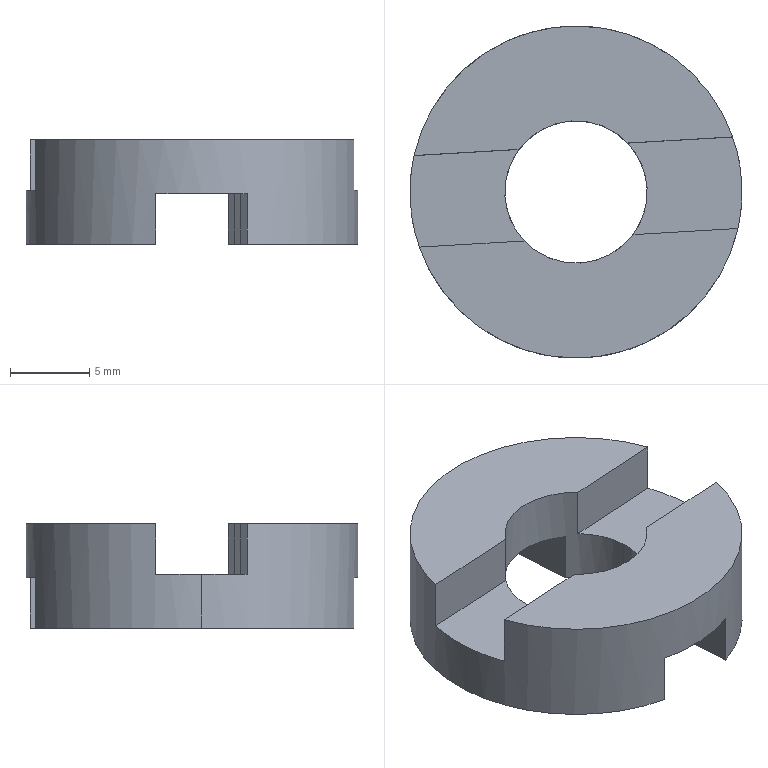Component | SolidWorks | MotorAssemblyWhen2-1_MCOCG20-8-10-1_MCOCG_spacer22-1 | 1 solid | 20 faces | box 21 x 21 x 6.6 mm | volume 1406 mm3 | plane 16 | cylinder 4 | commonest cylinder face diameters 21 x2 9 x2
STEP:
#1=COLOUR_RGB('',0.7922,0.8196,0.9333);
#2=FILL_AREA_STYLE_COLOUR('',#1);
#3=FILL_AREA_STYLE('',(#2));
#4=SURFACE_STYLE_FILL_AREA(#3);
#5=SURFACE_SIDE_STYLE('',(#4));
#6=SURFACE_STYLE_USAGE(.BOTH.,#5);
#7=PRESENTATION_STYLE_ASSIGNMENT((#6));
#8=CARTESIAN_POINT('',(-1.831,4.945,-4.699));
#9=VERTEX_POINT('',#8);
#10=CARTESIAN_POINT('',(-1.556,5.359,-4.699));
#11=VERTEX_POINT('',#10);
#12=CARTESIAN_POINT('',(-1.969,5.335,-4.699));
#13=DIRECTION('',(0.,-0.,1.));
#14=DIRECTION('',(-0.9983,-0.05821,0.));
#15=AXIS2_PLACEMENT_3D('',#12,#13,#14);
#16=CIRCLE('',#15,0.4134);
#17=EDGE_CURVE('',#9,#11,#16,.T.);
#18=ORIENTED_EDGE('',*,*,#17,.T.);
#19=CARTESIAN_POINT('',(-1.556,5.359,-4.565));
#20=VERTEX_POINT('',#19);
#21=CARTESIAN_POINT('',(-1.556,5.359,-4.699));
#22=DIRECTION('',(0.,-0.,1.));
#23=VECTOR('',#22,39.37);
#24=LINE('',#21,#23);
#25=EDGE_CURVE('',#11,#20,#24,.T.);
#26=ORIENTED_EDGE('',*,*,#25,.T.);
#27=CARTESIAN_POINT('',(-1.565,5.244,-4.565));
#28=VERTEX_POINT('',#27);
#29=CARTESIAN_POINT('',(-1.969,5.335,-4.565));
#30=DIRECTION('',(-0.,0.,-1.));
#31=DIRECTION('',(-0.9983,-0.05821,0.));
#32=AXIS2_PLACEMENT_3D('',#29,#30,#31);
#33=CIRCLE('',#32,0.4134);
#34=EDGE_CURVE('',#20,#28,#33,.T.);
#35=ORIENTED_EDGE('',*,*,#34,.T.);
#36=CARTESIAN_POINT('',(-1.565,5.244,-4.439));
#37=VERTEX_POINT('',#36);
#38=CARTESIAN_POINT('',(-1.565,5.244,-4.699));
#39=DIRECTION('',(0.,-0.,1.));
#40=VECTOR('',#39,39.37);
#41=LINE('',#38,#40);
#42=EDGE_CURVE('',#28,#37,#41,.T.);
#43=ORIENTED_EDGE('',*,*,#42,.T.);
#44=CARTESIAN_POINT('',(-2.358,5.198,-4.439));
#45=VERTEX_POINT('',#44);
#46=CARTESIAN_POINT('',(-1.969,5.335,-4.439));
#47=DIRECTION('',(-0.,0.,-1.));
#48=DIRECTION('',(-0.9983,-0.05821,0.));
#49=AXIS2_PLACEMENT_3D('',#46,#47,#48);
#50=CIRCLE('',#49,0.4134);
#51=EDGE_CURVE('',#37,#45,#50,.T.);
#52=ORIENTED_EDGE('',*,*,#51,.T.);
#53=CARTESIAN_POINT('',(-2.358,5.198,-4.565));
#54=VERTEX_POINT('',#53);
#55=CARTESIAN_POINT('',(-2.358,5.198,-4.699));
#56=DIRECTION('',(-0.,0.,-1.));
#57=VECTOR('',#56,39.37);
#58=LINE('',#55,#57);
#59=EDGE_CURVE('',#45,#54,#58,.T.);
#60=ORIENTED_EDGE('',*,*,#59,.T.);
#61=CARTESIAN_POINT('',(-2.381,5.311,-4.565));
#62=VERTEX_POINT('',#61);
#63=CARTESIAN_POINT('',(-1.969,5.335,-4.565));
#64=DIRECTION('',(-0.,0.,-1.));
#65=DIRECTION('',(-0.9983,-0.05821,0.));
#66=AXIS2_PLACEMENT_3D('',#63,#64,#65);
#67=CIRCLE('',#66,0.4134);
#68=EDGE_CURVE('',#54,#62,#67,.T.);
#69=ORIENTED_EDGE('',*,*,#68,.T.);
#70=CARTESIAN_POINT('',(-2.381,5.311,-4.699));
#71=VERTEX_POINT('',#70);
#72=CARTESIAN_POINT('',(-2.381,5.311,-4.699));
#73=DIRECTION('',(0.,-0.,1.));
#74=VECTOR('',#73,39.37);
#75=LINE('',#72,#74);
#76=EDGE_CURVE('',#71,#62,#75,.T.);
#77=ORIENTED_EDGE('',*,*,#76,.F.);
#78=CARTESIAN_POINT('',(-2.059,4.931,-4.699));
#79=VERTEX_POINT('',#78);
#80=CARTESIAN_POINT('',(-1.969,5.335,-4.699));
#81=DIRECTION('',(0.,-0.,1.));
#82=DIRECTION('',(-0.9983,-0.05821,0.));
#83=AXIS2_PLACEMENT_3D('',#80,#81,#82);
#84=CIRCLE('',#83,0.4134);
#85=EDGE_CURVE('',#71,#79,#84,.T.);
#86=ORIENTED_EDGE('',*,*,#85,.T.);
#87=CARTESIAN_POINT('',(-2.059,4.931,-4.573));
#88=VERTEX_POINT('',#87);
#89=CARTESIAN_POINT('',(-2.059,4.931,-4.699));
#90=DIRECTION('',(0.,-0.,1.));
#91=VECTOR('',#90,39.37);
#92=LINE('',#89,#91);
#93=EDGE_CURVE('',#79,#88,#92,.T.);
#94=ORIENTED_EDGE('',*,*,#93,.T.);
#95=CARTESIAN_POINT('',(-1.831,4.945,-4.573));
#96=VERTEX_POINT('',#95);
#97=CARTESIAN_POINT('',(-1.969,5.335,-4.573));
#98=DIRECTION('',(0.,-0.,1.));
#99=DIRECTION('',(-0.9983,-0.05821,0.));
#100=AXIS2_PLACEMENT_3D('',#97,#98,#99);
#101=CIRCLE('',#100,0.4134);
#102=EDGE_CURVE('',#88,#96,#101,.T.);
#103=ORIENTED_EDGE('',*,*,#102,.T.);
#104=CARTESIAN_POINT('',(-1.831,4.945,-4.699));
#105=DIRECTION('',(-0.,0.,-1.));
#106=VECTOR('',#105,39.37);
#107=LINE('',#104,#106);
#108=EDGE_CURVE('',#96,#9,#107,.T.);
#109=ORIENTED_EDGE('',*,*,#108,.T.);
#110=EDGE_LOOP('',(#18,#26,#35,#43,#52,#60,#69,#77,#86,#94,#103,#109));
#111=FACE_OUTER_BOUND('',#110,.T.);
#112=CARTESIAN_POINT('',(-1.969,5.335,-4.699));
#113=DIRECTION('',(0.,-0.,1.));
#114=DIRECTION('',(-0.9983,-0.05821,0.));
#115=AXIS2_PLACEMENT_3D('',#112,#113,#114);
#116=CYLINDRICAL_SURFACE('',#115,0.4134);
#117=ADVANCED_FACE('',(#111),#116,.T.);
#118=CARTESIAN_POINT('',(-1.862,5.477,-4.699));
#119=VERTEX_POINT('',#118);
#120=CARTESIAN_POINT('',(-1.792,5.345,-4.699));
#121=VERTEX_POINT('',#120);
#122=CARTESIAN_POINT('',(-1.969,5.335,-4.699));
#123=DIRECTION('',(-0.,0.,-1.));
#124=DIRECTION('',(-0.9983,-0.05821,0.));
#125=AXIS2_PLACEMENT_3D('',#122,#123,#124);
#126=CIRCLE('',#125,0.1772);
#127=EDGE_CURVE('',#119,#121,#126,.T.);
#128=ORIENTED_EDGE('',*,*,#127,.T.);
#129=CARTESIAN_POINT('',(-1.792,5.345,-4.565));
#130=VERTEX_POINT('',#129);
#131=CARTESIAN_POINT('',(-1.792,5.345,-4.699));
#132=DIRECTION('',(0.,-0.,1.));
#133=VECTOR('',#132,39.37);
#134=LINE('',#131,#133);
#135=EDGE_CURVE('',#121,#130,#134,.T.);
#136=ORIENTED_EDGE('',*,*,#135,.T.);
#137=CARTESIAN_POINT('',(-1.84,5.457,-4.565));
#138=VERTEX_POINT('',#137);
#139=CARTESIAN_POINT('',(-1.969,5.335,-4.565));
#140=DIRECTION('',(0.,-0.,1.));
#141=DIRECTION('',(-0.9983,-0.05821,0.));
#142=AXIS2_PLACEMENT_3D('',#139,#140,#141);
#143=CIRCLE('',#142,0.1772);
#144=EDGE_CURVE('',#130,#138,#143,.T.);
#145=ORIENTED_EDGE('',*,*,#144,.T.);
#146=CARTESIAN_POINT('',(-1.84,5.457,-4.439));
#147=VERTEX_POINT('',#146);
#148=CARTESIAN_POINT('',(-1.84,5.457,-4.439));
#149=DIRECTION('',(0.,-0.,1.));
#150=VECTOR('',#149,39.37);
#151=LINE('',#148,#150);
#152=EDGE_CURVE('',#138,#147,#151,.T.);
#153=ORIENTED_EDGE('',*,*,#152,.T.);
#154=CARTESIAN_POINT('',(-2.11,5.441,-4.439));
#155=VERTEX_POINT('',#154);
#156=CARTESIAN_POINT('',(-1.969,5.335,-4.439));
#157=DIRECTION('',(0.,-0.,1.));
#158=DIRECTION('',(-0.9983,-0.05821,0.));
#159=AXIS2_PLACEMENT_3D('',#156,#157,#158);
#160=CIRCLE('',#159,0.1772);
#161=EDGE_CURVE('',#147,#155,#160,.T.);
#162=ORIENTED_EDGE('',*,*,#161,.T.);
#163=CARTESIAN_POINT('',(-2.11,5.441,-4.565));
#164=VERTEX_POINT('',#163);
#165=CARTESIAN_POINT('',(-2.11,5.441,-4.439));
#166=DIRECTION('',(-0.,0.,-1.));
#167=VECTOR('',#166,39.37);
#168=LINE('',#165,#167);
#169=EDGE_CURVE('',#155,#164,#168,.T.);
#170=ORIENTED_EDGE('',*,*,#169,.T.);
#171=CARTESIAN_POINT('',(-2.145,5.324,-4.565));
#172=VERTEX_POINT('',#171);
#173=CARTESIAN_POINT('',(-1.969,5.335,-4.565));
#174=DIRECTION('',(0.,-0.,1.));
#175=DIRECTION('',(-0.9983,-0.05821,0.));
#176=AXIS2_PLACEMENT_3D('',#173,#174,#175);
#177=CIRCLE('',#176,0.1772);
#178=EDGE_CURVE('',#164,#172,#177,.T.);
#179=ORIENTED_EDGE('',*,*,#178,.T.);
#180=CARTESIAN_POINT('',(-2.145,5.324,-4.699));
#181=VERTEX_POINT('',#180);
#182=CARTESIAN_POINT('',(-2.145,5.324,-4.699));
#183=DIRECTION('',(0.,-0.,1.));
#184=VECTOR('',#183,39.37);
#185=LINE('',#182,#184);
#186=EDGE_CURVE('',#181,#172,#185,.T.);
#187=ORIENTED_EDGE('',*,*,#186,.F.);
#188=CARTESIAN_POINT('',(-2.09,5.463,-4.699));
#189=VERTEX_POINT('',#188);
#190=CARTESIAN_POINT('',(-1.969,5.335,-4.699));
#191=DIRECTION('',(-0.,0.,-1.));
#192=DIRECTION('',(-0.9983,-0.05821,0.));
#193=AXIS2_PLACEMENT_3D('',#190,#191,#192);
#194=CIRCLE('',#193,0.1772);
#195=EDGE_CURVE('',#181,#189,#194,.T.);
#196=ORIENTED_EDGE('',*,*,#195,.T.);
#197=CARTESIAN_POINT('',(-2.09,5.463,-4.573));
#198=VERTEX_POINT('',#197);
#199=CARTESIAN_POINT('',(-2.09,5.463,-4.573));
#200=DIRECTION('',(0.,-0.,1.));
#201=VECTOR('',#200,39.37);
#202=LINE('',#199,#201);
#203=EDGE_CURVE('',#189,#198,#202,.T.);
#204=ORIENTED_EDGE('',*,*,#203,.T.);
#205=CARTESIAN_POINT('',(-1.862,5.477,-4.573));
#206=VERTEX_POINT('',#205);
#207=CARTESIAN_POINT('',(-1.969,5.335,-4.573));
#208=DIRECTION('',(-0.,0.,-1.));
#209=DIRECTION('',(-0.9983,-0.05821,0.));
#210=AXIS2_PLACEMENT_3D('',#207,#208,#209);
#211=CIRCLE('',#210,0.1772);
#212=EDGE_CURVE('',#198,#206,#211,.T.);
#213=ORIENTED_EDGE('',*,*,#212,.T.);
#214=CARTESIAN_POINT('',(-1.862,5.477,-4.699));
#215=DIRECTION('',(-0.,0.,-1.));
#216=VECTOR('',#215,39.37);
#217=LINE('',#214,#216);
#218=EDGE_CURVE('',#206,#119,#217,.T.);
#219=ORIENTED_EDGE('',*,*,#218,.T.);
#220=EDGE_LOOP('',(#128,#136,#145,#153,#162,#170,#179,#187,#196,#204,#213,#219));
#221=FACE_OUTER_BOUND('',#220,.T.);
#222=CARTESIAN_POINT('',(-1.969,5.335,-4.699));
#223=DIRECTION('',(0.,-0.,1.));
#224=DIRECTION('',(-0.9983,-0.05821,0.));
#225=AXIS2_PLACEMENT_3D('',#222,#223,#224);
#226=CYLINDRICAL_SURFACE('',#225,0.1772);
#227=ADVANCED_FACE('',(#221),#226,.F.);
#228=ORIENTED_EDGE('',*,*,#25,.F.);
#229=CARTESIAN_POINT('',(-1.878,5.738,-4.699));
#230=VERTEX_POINT('',#229);
#231=CARTESIAN_POINT('',(-1.969,5.335,-4.699));
#232=DIRECTION('',(0.,-0.,1.));
#233=DIRECTION('',(-0.9983,-0.05821,0.));
#234=AXIS2_PLACEMENT_3D('',#231,#232,#233);
#235=CIRCLE('',#234,0.4134);
#236=EDGE_CURVE('',#11,#230,#235,.T.);
#237=ORIENTED_EDGE('',*,*,#236,.T.);
#238=CARTESIAN_POINT('',(-1.878,5.738,-4.573));
#239=VERTEX_POINT('',#238);
#240=CARTESIAN_POINT('',(-1.878,5.738,-4.699));
#241=DIRECTION('',(0.,-0.,1.));
#242=VECTOR('',#241,39.37);
#243=LINE('',#240,#242);
#244=EDGE_CURVE('',#230,#239,#243,.T.);
#245=ORIENTED_EDGE('',*,*,#244,.T.);
#246=CARTESIAN_POINT('',(-2.106,5.725,-4.573));
#247=VERTEX_POINT('',#246);
#248=CARTESIAN_POINT('',(-1.969,5.335,-4.573));
#249=DIRECTION('',(0.,-0.,1.));
#250=DIRECTION('',(-0.9983,-0.05821,0.));
#251=AXIS2_PLACEMENT_3D('',#248,#249,#250);
#252=CIRCLE('',#251,0.4134);
#253=EDGE_CURVE('',#239,#247,#252,.T.);
#254=ORIENTED_EDGE('',*,*,#253,.T.);
#255=CARTESIAN_POINT('',(-2.106,5.725,-4.699));
#256=VERTEX_POINT('',#255);
#257=CARTESIAN_POINT('',(-2.106,5.725,-4.699));
#258=DIRECTION('',(-0.,0.,-1.));
#259=VECTOR('',#258,39.37);
#260=LINE('',#257,#259);
#261=EDGE_CURVE('',#247,#256,#260,.T.);
#262=ORIENTED_EDGE('',*,*,#261,.T.);
#263=CARTESIAN_POINT('',(-1.969,5.335,-4.699));
#264=DIRECTION('',(0.,-0.,1.));
#265=DIRECTION('',(-0.9983,-0.05821,0.));
#266=AXIS2_PLACEMENT_3D('',#263,#264,#265);
#267=CIRCLE('',#266,0.4134);
#268=EDGE_CURVE('',#256,#71,#267,.T.);
#269=ORIENTED_EDGE('',*,*,#268,.T.);
#270=ORIENTED_EDGE('',*,*,#76,.T.);
#271=CARTESIAN_POINT('',(-2.372,5.426,-4.565));
#272=VERTEX_POINT('',#271);
#273=CARTESIAN_POINT('',(-1.969,5.335,-4.565));
#274=DIRECTION('',(-0.,0.,-1.));
#275=DIRECTION('',(-0.9983,-0.05821,0.));
#276=AXIS2_PLACEMENT_3D('',#273,#274,#275);
#277=CIRCLE('',#276,0.4134);
#278=EDGE_CURVE('',#62,#272,#277,.T.);
#279=ORIENTED_EDGE('',*,*,#278,.T.);
#280=CARTESIAN_POINT('',(-2.372,5.426,-4.439));
#281=VERTEX_POINT('',#280);
#282=CARTESIAN_POINT('',(-2.372,5.426,-4.699));
#283=DIRECTION('',(0.,-0.,1.));
#284=VECTOR('',#283,39.37);
#285=LINE('',#282,#284);
#286=EDGE_CURVE('',#272,#281,#285,.T.);
#287=ORIENTED_EDGE('',*,*,#286,.T.);
#288=CARTESIAN_POINT('',(-1.579,5.472,-4.439));
#289=VERTEX_POINT('',#288);
#290=CARTESIAN_POINT('',(-1.969,5.335,-4.439));
#291=DIRECTION('',(-0.,0.,-1.));
#292=DIRECTION('',(-0.9983,-0.05821,0.));
#293=AXIS2_PLACEMENT_3D('',#290,#291,#292);
#294=CIRCLE('',#293,0.4134);
#295=EDGE_CURVE('',#281,#289,#294,.T.);
#296=ORIENTED_EDGE('',*,*,#295,.T.);
#297=CARTESIAN_POINT('',(-1.579,5.472,-4.565));
#298=VERTEX_POINT('',#297);
#299=CARTESIAN_POINT('',(-1.579,5.472,-4.699));
#300=DIRECTION('',(-0.,0.,-1.));
#301=VECTOR('',#300,39.37);
#302=LINE('',#299,#301);
#303=EDGE_CURVE('',#289,#298,#302,.T.);
#304=ORIENTED_EDGE('',*,*,#303,.T.);
#305=CARTESIAN_POINT('',(-1.969,5.335,-4.565));
#306=DIRECTION('',(-0.,0.,-1.));
#307=DIRECTION('',(-0.9983,-0.05821,0.));
#308=AXIS2_PLACEMENT_3D('',#305,#306,#307);
#309=CIRCLE('',#308,0.4134);
#310=EDGE_CURVE('',#298,#20,#309,.T.);
#311=ORIENTED_EDGE('',*,*,#310,.T.);
#312=EDGE_LOOP('',(#228,#237,#245,#254,#262,#269,#270,#279,#287,#296,#304,#311));
#313=FACE_OUTER_BOUND('',#312,.T.);
#314=CARTESIAN_POINT('',(-1.969,5.335,-4.699));
#315=DIRECTION('',(0.,-0.,1.));
#316=DIRECTION('',(-0.9983,-0.05821,0.));
#317=AXIS2_PLACEMENT_3D('',#314,#315,#316);
#318=CYLINDRICAL_SURFACE('',#317,0.4134);
#319=ADVANCED_FACE('',(#313),#318,.T.);
#320=CARTESIAN_POINT('',(-1.562,5.473,-4.565));
#321=DIRECTION('',(0.9983,0.05821,0.));
#322=VECTOR('',#321,39.37);
#323=LINE('',#320,#322);
#324=EDGE_CURVE('',#138,#298,#323,.T.);
#325=ORIENTED_EDGE('',*,*,#324,.F.);
#326=ORIENTED_EDGE('',*,*,#144,.F.);
#327=CARTESIAN_POINT('',(-1.827,5.229,-4.565));
#328=VERTEX_POINT('',#327);
#329=CARTESIAN_POINT('',(-1.969,5.335,-4.565));
#330=DIRECTION('',(0.,-0.,1.));
#331=DIRECTION('',(-0.9983,-0.05821,0.));
#332=AXIS2_PLACEMENT_3D('',#329,#330,#331);
#333=CIRCLE('',#332,0.1772);
#334=EDGE_CURVE('',#328,#130,#333,.T.);
#335=ORIENTED_EDGE('',*,*,#334,.F.);
#336=CARTESIAN_POINT('',(-1.549,5.245,-4.565));
#337=DIRECTION('',(-0.9983,-0.05821,-0.));
#338=VECTOR('',#337,39.37);
#339=LINE('',#336,#338);
#340=EDGE_CURVE('',#28,#328,#339,.T.);
#341=ORIENTED_EDGE('',*,*,#340,.F.);
#342=ORIENTED_EDGE('',*,*,#34,.F.);
#343=ORIENTED_EDGE('',*,*,#310,.F.);
#344=EDGE_LOOP('',(#325,#326,#335,#341,#342,#343));
#345=FACE_OUTER_BOUND('',#344,.T.);
#346=CARTESIAN_POINT('',(-1.562,5.473,-4.565));
#347=DIRECTION('',(0.,0.,-1.));
#348=DIRECTION('',(0.9983,0.05821,0.));
#349=AXIS2_PLACEMENT_3D('',#346,#347,#348);
#350=PLANE('',#349);
#351=ADVANCED_FACE('',(#345),#350,.F.);
#352=ORIENTED_EDGE('',*,*,#152,.F.);
#353=ORIENTED_EDGE('',*,*,#324,.T.);
#354=ORIENTED_EDGE('',*,*,#303,.F.);
#355=CARTESIAN_POINT('',(-1.562,5.473,-4.439));
#356=DIRECTION('',(0.9983,0.05821,0.));
#357=VECTOR('',#356,39.37);
#358=LINE('',#355,#357);
#359=EDGE_CURVE('',#147,#289,#358,.T.);
#360=ORIENTED_EDGE('',*,*,#359,.F.);
#361=EDGE_LOOP('',(#352,#353,#354,#360));
#362=FACE_OUTER_BOUND('',#361,.T.);
#363=CARTESIAN_POINT('',(-1.562,5.473,-4.439));
#364=DIRECTION('',(-0.05821,0.9983,0.));
#365=DIRECTION('',(0.9983,0.05821,0.));
#366=AXIS2_PLACEMENT_3D('',#363,#364,#365);
#367=PLANE('',#366);
#368=ADVANCED_FACE('',(#362),#367,.F.);
#369=CARTESIAN_POINT('',(-1.975,5.449,-4.439));
#370=DIRECTION('',(-0.9983,-0.05821,-0.));
#371=VECTOR('',#370,39.37);
#372=LINE('',#369,#371);
#373=EDGE_CURVE('',#155,#281,#372,.T.);
#374=ORIENTED_EDGE('',*,*,#373,.F.);
#375=ORIENTED_EDGE('',*,*,#161,.F.);
#376=ORIENTED_EDGE('',*,*,#359,.T.);
#377=ORIENTED_EDGE('',*,*,#295,.F.);
#378=EDGE_LOOP('',(#374,#375,#376,#377));
#379=FACE_OUTER_BOUND('',#378,.T.);
#380=CARTESIAN_POINT('',(-1.944,4.922,-4.439));
#381=DIRECTION('',(0.,0.,-1.));
#382=DIRECTION('',(0.9983,0.05821,0.));
#383=AXIS2_PLACEMENT_3D('',#380,#381,#382);
#384=PLANE('',#383);
#385=ADVANCED_FACE('',(#379),#384,.F.);
#386=ORIENTED_EDGE('',*,*,#169,.F.);
#387=ORIENTED_EDGE('',*,*,#373,.T.);
#388=ORIENTED_EDGE('',*,*,#286,.F.);
#389=CARTESIAN_POINT('',(-1.562,5.473,-4.565));
#390=DIRECTION('',(-0.9983,-0.05821,-0.));
#391=VECTOR('',#390,39.37);
#392=LINE('',#389,#391);
#393=EDGE_CURVE('',#164,#272,#392,.T.);
#394=ORIENTED_EDGE('',*,*,#393,.F.);
#395=EDGE_LOOP('',(#386,#387,#388,#394));
#396=FACE_OUTER_BOUND('',#395,.T.);
#397=CARTESIAN_POINT('',(-1.562,5.473,-4.439));
#398=DIRECTION('',(-0.05821,0.9983,0.));
#399=DIRECTION('',(0.9983,0.05821,0.));
#400=AXIS2_PLACEMENT_3D('',#397,#398,#399);
#401=PLANE('',#400);
#402=ADVANCED_FACE('',(#396),#401,.F.);
#403=ORIENTED_EDGE('',*,*,#178,.F.);
#404=ORIENTED_EDGE('',*,*,#393,.T.);
#405=ORIENTED_EDGE('',*,*,#278,.F.);
#406=ORIENTED_EDGE('',*,*,#68,.F.);
#407=CARTESIAN_POINT('',(-2.097,5.213,-4.565));
#408=VERTEX_POINT('',#407);
#409=CARTESIAN_POINT('',(-1.549,5.245,-4.565));
#410=DIRECTION('',(-0.9983,-0.05821,-0.));
#411=VECTOR('',#410,39.37);
#412=LINE('',#409,#411);
#413=EDGE_CURVE('',#408,#54,#412,.T.);
#414=ORIENTED_EDGE('',*,*,#413,.F.);
#415=CARTESIAN_POINT('',(-1.969,5.335,-4.565));
#416=DIRECTION('',(0.,-0.,1.));
#417=DIRECTION('',(-0.9983,-0.05821,0.));
#418=AXIS2_PLACEMENT_3D('',#415,#416,#417);
#419=CIRCLE('',#418,0.1772);
#420=EDGE_CURVE('',#172,#408,#419,.T.);
#421=ORIENTED_EDGE('',*,*,#420,.F.);
#422=EDGE_LOOP('',(#403,#404,#405,#406,#414,#421));
#423=FACE_OUTER_BOUND('',#422,.T.);
#424=CARTESIAN_POINT('',(-1.562,5.473,-4.565));
#425=DIRECTION('',(0.,0.,-1.));
#426=DIRECTION('',(0.9983,0.05821,0.));
#427=AXIS2_PLACEMENT_3D('',#424,#425,#426);
#428=PLANE('',#427);
#429=ADVANCED_FACE('',(#423),#428,.F.);
#430=CARTESIAN_POINT('',(-2.072,5.151,-4.699));
#431=DIRECTION('',(-0.05821,0.9983,0.));
#432=VECTOR('',#431,39.37);
#433=LINE('',#430,#432);
#434=EDGE_CURVE('',#189,#256,#433,.T.);
#435=ORIENTED_EDGE('',*,*,#434,.F.);
#436=ORIENTED_EDGE('',*,*,#195,.F.);
#437=CARTESIAN_POINT('',(-2.075,5.193,-4.699));
#438=VERTEX_POINT('',#437);
#439=CARTESIAN_POINT('',(-1.969,5.335,-4.699));
#440=DIRECTION('',(-0.,0.,-1.));
#441=DIRECTION('',(-0.9983,-0.05821,0.));
#442=AXIS2_PLACEMENT_3D('',#439,#440,#441);
#443=CIRCLE('',#442,0.1772);
#444=EDGE_CURVE('',#438,#181,#443,.T.);
#445=ORIENTED_EDGE('',*,*,#444,.F.);
#446=CARTESIAN_POINT('',(-2.072,5.151,-4.699));
#447=DIRECTION('',(-0.05821,0.9983,0.));
#448=VECTOR('',#447,39.37);
#449=LINE('',#446,#448);
#450=EDGE_CURVE('',#79,#438,#449,.T.);
#451=ORIENTED_EDGE('',*,*,#450,.F.);
#452=ORIENTED_EDGE('',*,*,#85,.F.);
#453=ORIENTED_EDGE('',*,*,#268,.F.);
#454=EDGE_LOOP('',(#435,#436,#445,#451,#452,#453));
#455=FACE_OUTER_BOUND('',#454,.T.);
#456=CARTESIAN_POINT('',(-1.958,5.158,-4.699));
#457=DIRECTION('',(-0.,-0.,1.));
#458=DIRECTION('',(-0.9983,-0.05821,-0.));
#459=AXIS2_PLACEMENT_3D('',#456,#457,#458);
#460=PLANE('',#459);
#461=ADVANCED_FACE('',(#455),#460,.F.);
#462=ORIENTED_EDGE('',*,*,#203,.F.);
#463=ORIENTED_EDGE('',*,*,#434,.T.);
#464=ORIENTED_EDGE('',*,*,#261,.F.);
#465=CARTESIAN_POINT('',(-2.107,5.741,-4.573));
#466=DIRECTION('',(-0.05821,0.9983,0.));
#467=VECTOR('',#466,39.37);
#468=LINE('',#465,#467);
#469=EDGE_CURVE('',#198,#247,#468,.T.);
#470=ORIENTED_EDGE('',*,*,#469,.F.);
#471=EDGE_LOOP('',(#462,#463,#464,#470));
#472=FACE_OUTER_BOUND('',#471,.T.);
#473=CARTESIAN_POINT('',(-2.107,5.741,-4.573));
#474=DIRECTION('',(-0.9983,-0.05821,-0.));
#475=DIRECTION('',(-0.,0.,-1.));
#476=AXIS2_PLACEMENT_3D('',#473,#474,#475);
#477=PLANE('',#476);
#478=ADVANCED_FACE('',(#472),#477,.F.);
#479=ORIENTED_EDGE('',*,*,#212,.F.);
#480=ORIENTED_EDGE('',*,*,#469,.T.);
#481=ORIENTED_EDGE('',*,*,#253,.F.);
#482=CARTESIAN_POINT('',(-1.879,5.754,-4.573));
#483=DIRECTION('',(-0.05821,0.9983,0.));
#484=VECTOR('',#483,39.37);
#485=LINE('',#482,#484);
#486=EDGE_CURVE('',#206,#239,#485,.T.);
#487=ORIENTED_EDGE('',*,*,#486,.F.);
#488=EDGE_LOOP('',(#479,#480,#481,#487));
#489=FACE_OUTER_BOUND('',#488,.T.);
#490=CARTESIAN_POINT('',(-1.879,5.754,-4.573));
#491=DIRECTION('',(-0.,-0.,1.));
#492=DIRECTION('',(-0.9983,-0.05821,-0.));
#493=AXIS2_PLACEMENT_3D('',#490,#491,#492);
#494=PLANE('',#493);
#495=ADVANCED_FACE('',(#489),#494,.F.);
#496=ORIENTED_EDGE('',*,*,#218,.F.);
#497=ORIENTED_EDGE('',*,*,#486,.T.);
#498=ORIENTED_EDGE('',*,*,#244,.F.);
#499=CARTESIAN_POINT('',(-1.879,5.754,-4.699));
#500=DIRECTION('',(-0.05821,0.9983,0.));
#501=VECTOR('',#500,39.37);
#502=LINE('',#499,#501);
#503=EDGE_CURVE('',#119,#230,#502,.T.);
#504=ORIENTED_EDGE('',*,*,#503,.F.);
#505=EDGE_LOOP('',(#496,#497,#498,#504));
#506=FACE_OUTER_BOUND('',#505,.T.);
#507=CARTESIAN_POINT('',(-1.879,5.754,-4.699));
#508=DIRECTION('',(0.9983,0.05821,0.));
#509=DIRECTION('',(0.,-0.,1.));
#510=AXIS2_PLACEMENT_3D('',#507,#508,#509);
#511=PLANE('',#510);
#512=ADVANCED_FACE('',(#506),#511,.F.);
#513=CARTESIAN_POINT('',(-1.847,5.206,-4.699));
#514=VERTEX_POINT('',#513);
#515=CARTESIAN_POINT('',(-1.844,5.164,-4.699));
#516=DIRECTION('',(0.05821,-0.9983,-0.));
#517=VECTOR('',#516,39.37);
#518=LINE('',#515,#517);
#519=EDGE_CURVE('',#514,#9,#518,.T.);
#520=ORIENTED_EDGE('',*,*,#519,.F.);
#521=CARTESIAN_POINT('',(-1.969,5.335,-4.699));
#522=DIRECTION('',(-0.,0.,-1.));
#523=DIRECTION('',(-0.9983,-0.05821,0.));
#524=AXIS2_PLACEMENT_3D('',#521,#522,#523);
#525=CIRCLE('',#524,0.1772);
#526=EDGE_CURVE('',#121,#514,#525,.T.);
#527=ORIENTED_EDGE('',*,*,#526,.F.);
#528=ORIENTED_EDGE('',*,*,#127,.F.);
#529=ORIENTED_EDGE('',*,*,#503,.T.);
#530=ORIENTED_EDGE('',*,*,#236,.F.);
#531=ORIENTED_EDGE('',*,*,#17,.F.);
#532=EDGE_LOOP('',(#520,#527,#528,#529,#530,#531));
#533=FACE_OUTER_BOUND('',#532,.T.);
#534=CARTESIAN_POINT('',(-1.958,5.158,-4.699));
#535=DIRECTION('',(-0.,-0.,1.));
#536=DIRECTION('',(-0.9983,-0.05821,-0.));
#537=AXIS2_PLACEMENT_3D('',#534,#535,#536);
#538=PLANE('',#537);
#539=ADVANCED_FACE('',(#533),#538,.F.);
#540=ORIENTED_EDGE('',*,*,#135,.F.);
#541=ORIENTED_EDGE('',*,*,#526,.T.);
#542=CARTESIAN_POINT('',(-1.847,5.206,-4.573));
#543=VERTEX_POINT('',#542);
#544=CARTESIAN_POINT('',(-1.847,5.206,-4.699));
#545=DIRECTION('',(-0.,0.,-1.));
#546=VECTOR('',#545,39.37);
#547=LINE('',#544,#546);
#548=EDGE_CURVE('',#543,#514,#547,.T.);
#549=ORIENTED_EDGE('',*,*,#548,.F.);
#550=CARTESIAN_POINT('',(-2.075,5.193,-4.573));
#551=VERTEX_POINT('',#550);
#552=CARTESIAN_POINT('',(-1.969,5.335,-4.573));
#553=DIRECTION('',(0.,-0.,1.));
#554=DIRECTION('',(-0.9983,-0.05821,0.));
#555=AXIS2_PLACEMENT_3D('',#552,#553,#554);
#556=CIRCLE('',#555,0.1772);
#557=EDGE_CURVE('',#551,#543,#556,.T.);
#558=ORIENTED_EDGE('',*,*,#557,.F.);
#559=CARTESIAN_POINT('',(-2.075,5.193,-4.699));
#560=DIRECTION('',(0.,-0.,1.));
#561=VECTOR('',#560,39.37);
#562=LINE('',#559,#561);
#563=EDGE_CURVE('',#438,#551,#562,.T.);
#564=ORIENTED_EDGE('',*,*,#563,.F.);
#565=ORIENTED_EDGE('',*,*,#444,.T.);
#566=ORIENTED_EDGE('',*,*,#186,.T.);
#567=ORIENTED_EDGE('',*,*,#420,.T.);
#568=CARTESIAN_POINT('',(-2.097,5.213,-4.439));
#569=VERTEX_POINT('',#568);
#570=CARTESIAN_POINT('',(-2.097,5.213,-4.699));
#571=DIRECTION('',(-0.,0.,-1.));
#572=VECTOR('',#571,39.37);
#573=LINE('',#570,#572);
#574=EDGE_CURVE('',#569,#408,#573,.T.);
#575=ORIENTED_EDGE('',*,*,#574,.F.);
#576=CARTESIAN_POINT('',(-1.827,5.229,-4.439));
#577=VERTEX_POINT('',#576);
#578=CARTESIAN_POINT('',(-1.969,5.335,-4.439));
#579=DIRECTION('',(-0.,0.,-1.));
#580=DIRECTION('',(-0.9983,-0.05821,0.));
#581=AXIS2_PLACEMENT_3D('',#578,#579,#580);
#582=CIRCLE('',#581,0.1772);
#583=EDGE_CURVE('',#577,#569,#582,.T.);
#584=ORIENTED_EDGE('',*,*,#583,.F.);
#585=CARTESIAN_POINT('',(-1.827,5.229,-4.699));
#586=DIRECTION('',(0.,-0.,1.));
#587=VECTOR('',#586,39.37);
#588=LINE('',#585,#587);
#589=EDGE_CURVE('',#328,#577,#588,.T.);
#590=ORIENTED_EDGE('',*,*,#589,.F.);
#591=ORIENTED_EDGE('',*,*,#334,.T.);
#592=EDGE_LOOP('',(#540,#541,#549,#558,#564,#565,#566,#567,#575,#584,#590,#591));
#593=FACE_OUTER_BOUND('',#592,.T.);
#594=CARTESIAN_POINT('',(-1.969,5.335,-4.699));
#595=DIRECTION('',(0.,-0.,1.));
#596=DIRECTION('',(-0.9983,-0.05821,0.));
#597=AXIS2_PLACEMENT_3D('',#594,#595,#596);
#598=CYLINDRICAL_SURFACE('',#597,0.1772);
#599=ADVANCED_FACE('',(#593),#598,.F.);
#600=ORIENTED_EDGE('',*,*,#589,.T.);
#601=CARTESIAN_POINT('',(-1.549,5.245,-4.439));
#602=DIRECTION('',(-0.9983,-0.05821,-0.));
#603=VECTOR('',#602,39.37);
#604=LINE('',#601,#603);
#605=EDGE_CURVE('',#37,#577,#604,.T.);
#606=ORIENTED_EDGE('',*,*,#605,.F.);
#607=ORIENTED_EDGE('',*,*,#42,.F.);
#608=ORIENTED_EDGE('',*,*,#340,.T.);
#609=EDGE_LOOP('',(#600,#606,#607,#608));
#610=FACE_OUTER_BOUND('',#609,.T.);
#611=CARTESIAN_POINT('',(-1.549,5.245,-4.565));
#612=DIRECTION('',(0.05821,-0.9983,-0.));
#613=DIRECTION('',(-0.9983,-0.05821,-0.));
#614=AXIS2_PLACEMENT_3D('',#611,#612,#613);
#615=PLANE('',#614);
#616=ADVANCED_FACE('',(#610),#615,.F.);
#617=ORIENTED_EDGE('',*,*,#574,.T.);
#618=ORIENTED_EDGE('',*,*,#413,.T.);
#619=ORIENTED_EDGE('',*,*,#59,.F.);
#620=CARTESIAN_POINT('',(-1.549,5.245,-4.439));
#621=DIRECTION('',(-0.9983,-0.05821,-0.));
#622=VECTOR('',#621,39.37);
#623=LINE('',#620,#622);
#624=EDGE_CURVE('',#569,#45,#623,.T.);
#625=ORIENTED_EDGE('',*,*,#624,.F.);
#626=EDGE_LOOP('',(#617,#618,#619,#625));
#627=FACE_OUTER_BOUND('',#626,.T.);
#628=CARTESIAN_POINT('',(-1.549,5.245,-4.565));
#629=DIRECTION('',(0.05821,-0.9983,-0.));
#630=DIRECTION('',(-0.9983,-0.05821,-0.));
#631=AXIS2_PLACEMENT_3D('',#628,#629,#630);
#632=PLANE('',#631);
#633=ADVANCED_FACE('',(#627),#632,.F.);
#634=ORIENTED_EDGE('',*,*,#548,.T.);
#635=ORIENTED_EDGE('',*,*,#519,.T.);
#636=ORIENTED_EDGE('',*,*,#108,.F.);
#637=CARTESIAN_POINT('',(-1.879,5.754,-4.573));
#638=DIRECTION('',(0.05821,-0.9983,-0.));
#639=VECTOR('',#638,39.37);
#640=LINE('',#637,#639);
#641=EDGE_CURVE('',#543,#96,#640,.T.);
#642=ORIENTED_EDGE('',*,*,#641,.F.);
#643=EDGE_LOOP('',(#634,#635,#636,#642));
#644=FACE_OUTER_BOUND('',#643,.T.);
#645=CARTESIAN_POINT('',(-1.879,5.754,-4.699));
#646=DIRECTION('',(0.9983,0.05821,0.));
#647=DIRECTION('',(0.,-0.,1.));
#648=AXIS2_PLACEMENT_3D('',#645,#646,#647);
#649=PLANE('',#648);
#650=ADVANCED_FACE('',(#644),#649,.F.);
#651=ORIENTED_EDGE('',*,*,#557,.T.);
#652=ORIENTED_EDGE('',*,*,#641,.T.);
#653=ORIENTED_EDGE('',*,*,#102,.F.);
#654=CARTESIAN_POINT('',(-2.107,5.741,-4.573));
#655=DIRECTION('',(0.05821,-0.9983,-0.));
#656=VECTOR('',#655,39.37);
#657=LINE('',#654,#656);
#658=EDGE_CURVE('',#551,#88,#657,.T.);
#659=ORIENTED_EDGE('',*,*,#658,.F.);
#660=EDGE_LOOP('',(#651,#652,#653,#659));
#661=FACE_OUTER_BOUND('',#660,.T.);
#662=CARTESIAN_POINT('',(-1.879,5.754,-4.573));
#663=DIRECTION('',(-0.,-0.,1.));
#664=DIRECTION('',(-0.9983,-0.05821,-0.));
#665=AXIS2_PLACEMENT_3D('',#662,#663,#664);
#666=PLANE('',#665);
#667=ADVANCED_FACE('',(#661),#666,.F.);
#668=ORIENTED_EDGE('',*,*,#563,.T.);
#669=ORIENTED_EDGE('',*,*,#658,.T.);
#670=ORIENTED_EDGE('',*,*,#93,.F.);
#671=ORIENTED_EDGE('',*,*,#450,.T.);
#672=EDGE_LOOP('',(#668,#669,#670,#671));
#673=FACE_OUTER_BOUND('',#672,.T.);
#674=CARTESIAN_POINT('',(-2.107,5.741,-4.573));
#675=DIRECTION('',(-0.9983,-0.05821,-0.));
#676=DIRECTION('',(-0.,0.,-1.));
#677=AXIS2_PLACEMENT_3D('',#674,#675,#676);
#678=PLANE('',#677);
#679=ADVANCED_FACE('',(#673),#678,.F.);
#680=ORIENTED_EDGE('',*,*,#605,.T.);
#681=ORIENTED_EDGE('',*,*,#583,.T.);
#682=ORIENTED_EDGE('',*,*,#624,.T.);
#683=ORIENTED_EDGE('',*,*,#51,.F.);
#684=EDGE_LOOP('',(#680,#681,#682,#683));
#685=FACE_OUTER_BOUND('',#684,.T.);
#686=CARTESIAN_POINT('',(-1.944,4.922,-4.439));
#687=DIRECTION('',(0.,0.,-1.));
#688=DIRECTION('',(0.9983,0.05821,0.));
#689=AXIS2_PLACEMENT_3D('',#686,#687,#688);
#690=PLANE('',#689);
#691=ADVANCED_FACE('',(#685),#690,.F.);
#692=CLOSED_SHELL('',(#117,#227,#319,#351,#368,#385,#402,#429,#461,#478,#495,#512,#539,#599,#616,#633,#650,#667,#679,#691));
#693=MANIFOLD_SOLID_BREP('',#692);
#694=STYLED_ITEM('',(#7),#693);
#695=PRESENTATION_LAYER_ASSIGNMENT('','',(#694));
#696=CARTESIAN_POINT('',(0.,0.,0.));
#697=DIRECTION('',(0.,0.,1.));
#698=DIRECTION('',(1.,0.,0.));
#699=AXIS2_PLACEMENT_3D('',#696,#697,#698);
#700=(LENGTH_UNIT()NAMED_UNIT(*)SI_UNIT($,.METRE.));
#701=LENGTH_MEASURE_WITH_UNIT(LENGTH_MEASURE(0.0254),#700);
#702=DIMENSIONAL_EXPONENTS(1.,0.,0.,0.,0.,0.,0.);
#703=(CONVERSION_BASED_UNIT('',#701)LENGTH_UNIT()NAMED_UNIT(#702));
#704=UNCERTAINTY_MEASURE_WITH_UNIT(LENGTH_MEASURE(0.00001),#703,'','');
#705=(NAMED_UNIT(*)PLANE_ANGLE_UNIT()SI_UNIT($,.RADIAN.));
#706=(NAMED_UNIT(*)SI_UNIT($,.STERADIAN.)SOLID_ANGLE_UNIT());
#707=(GEOMETRIC_REPRESENTATION_CONTEXT(3)GLOBAL_UNCERTAINTY_ASSIGNED_CONTEXT((#704))GLOBAL_UNIT_ASSIGNED_CONTEXT((#703,#705,#706))REPRESENTATION_CONTEXT('',''));
#708=ADVANCED_BREP_SHAPE_REPRESENTATION('',(#693,#699),#707);
#709=(LENGTH_UNIT()NAMED_UNIT(*)SI_UNIT($,.METRE.));
#710=LENGTH_MEASURE_WITH_UNIT(LENGTH_MEASURE(0.0254),#709);
#711=DIMENSIONAL_EXPONENTS(1.,0.,0.,0.,0.,0.,0.);
#712=(CONVERSION_BASED_UNIT('',#710)LENGTH_UNIT()NAMED_UNIT(#711));
#713=UNCERTAINTY_MEASURE_WITH_UNIT(LENGTH_MEASURE(0.00001),#712,'','');
#714=(NAMED_UNIT(*)PLANE_ANGLE_UNIT()SI_UNIT($,.RADIAN.));
#715=(NAMED_UNIT(*)SI_UNIT($,.STERADIAN.)SOLID_ANGLE_UNIT());
#716=(GEOMETRIC_REPRESENTATION_CONTEXT(3)GLOBAL_UNCERTAINTY_ASSIGNED_CONTEXT((#713))GLOBAL_UNIT_ASSIGNED_CONTEXT((#712,#714,#715))REPRESENTATION_CONTEXT('',''));
#717=MECHANICAL_DESIGN_GEOMETRIC_PRESENTATION_REPRESENTATION('',(#694),#716);